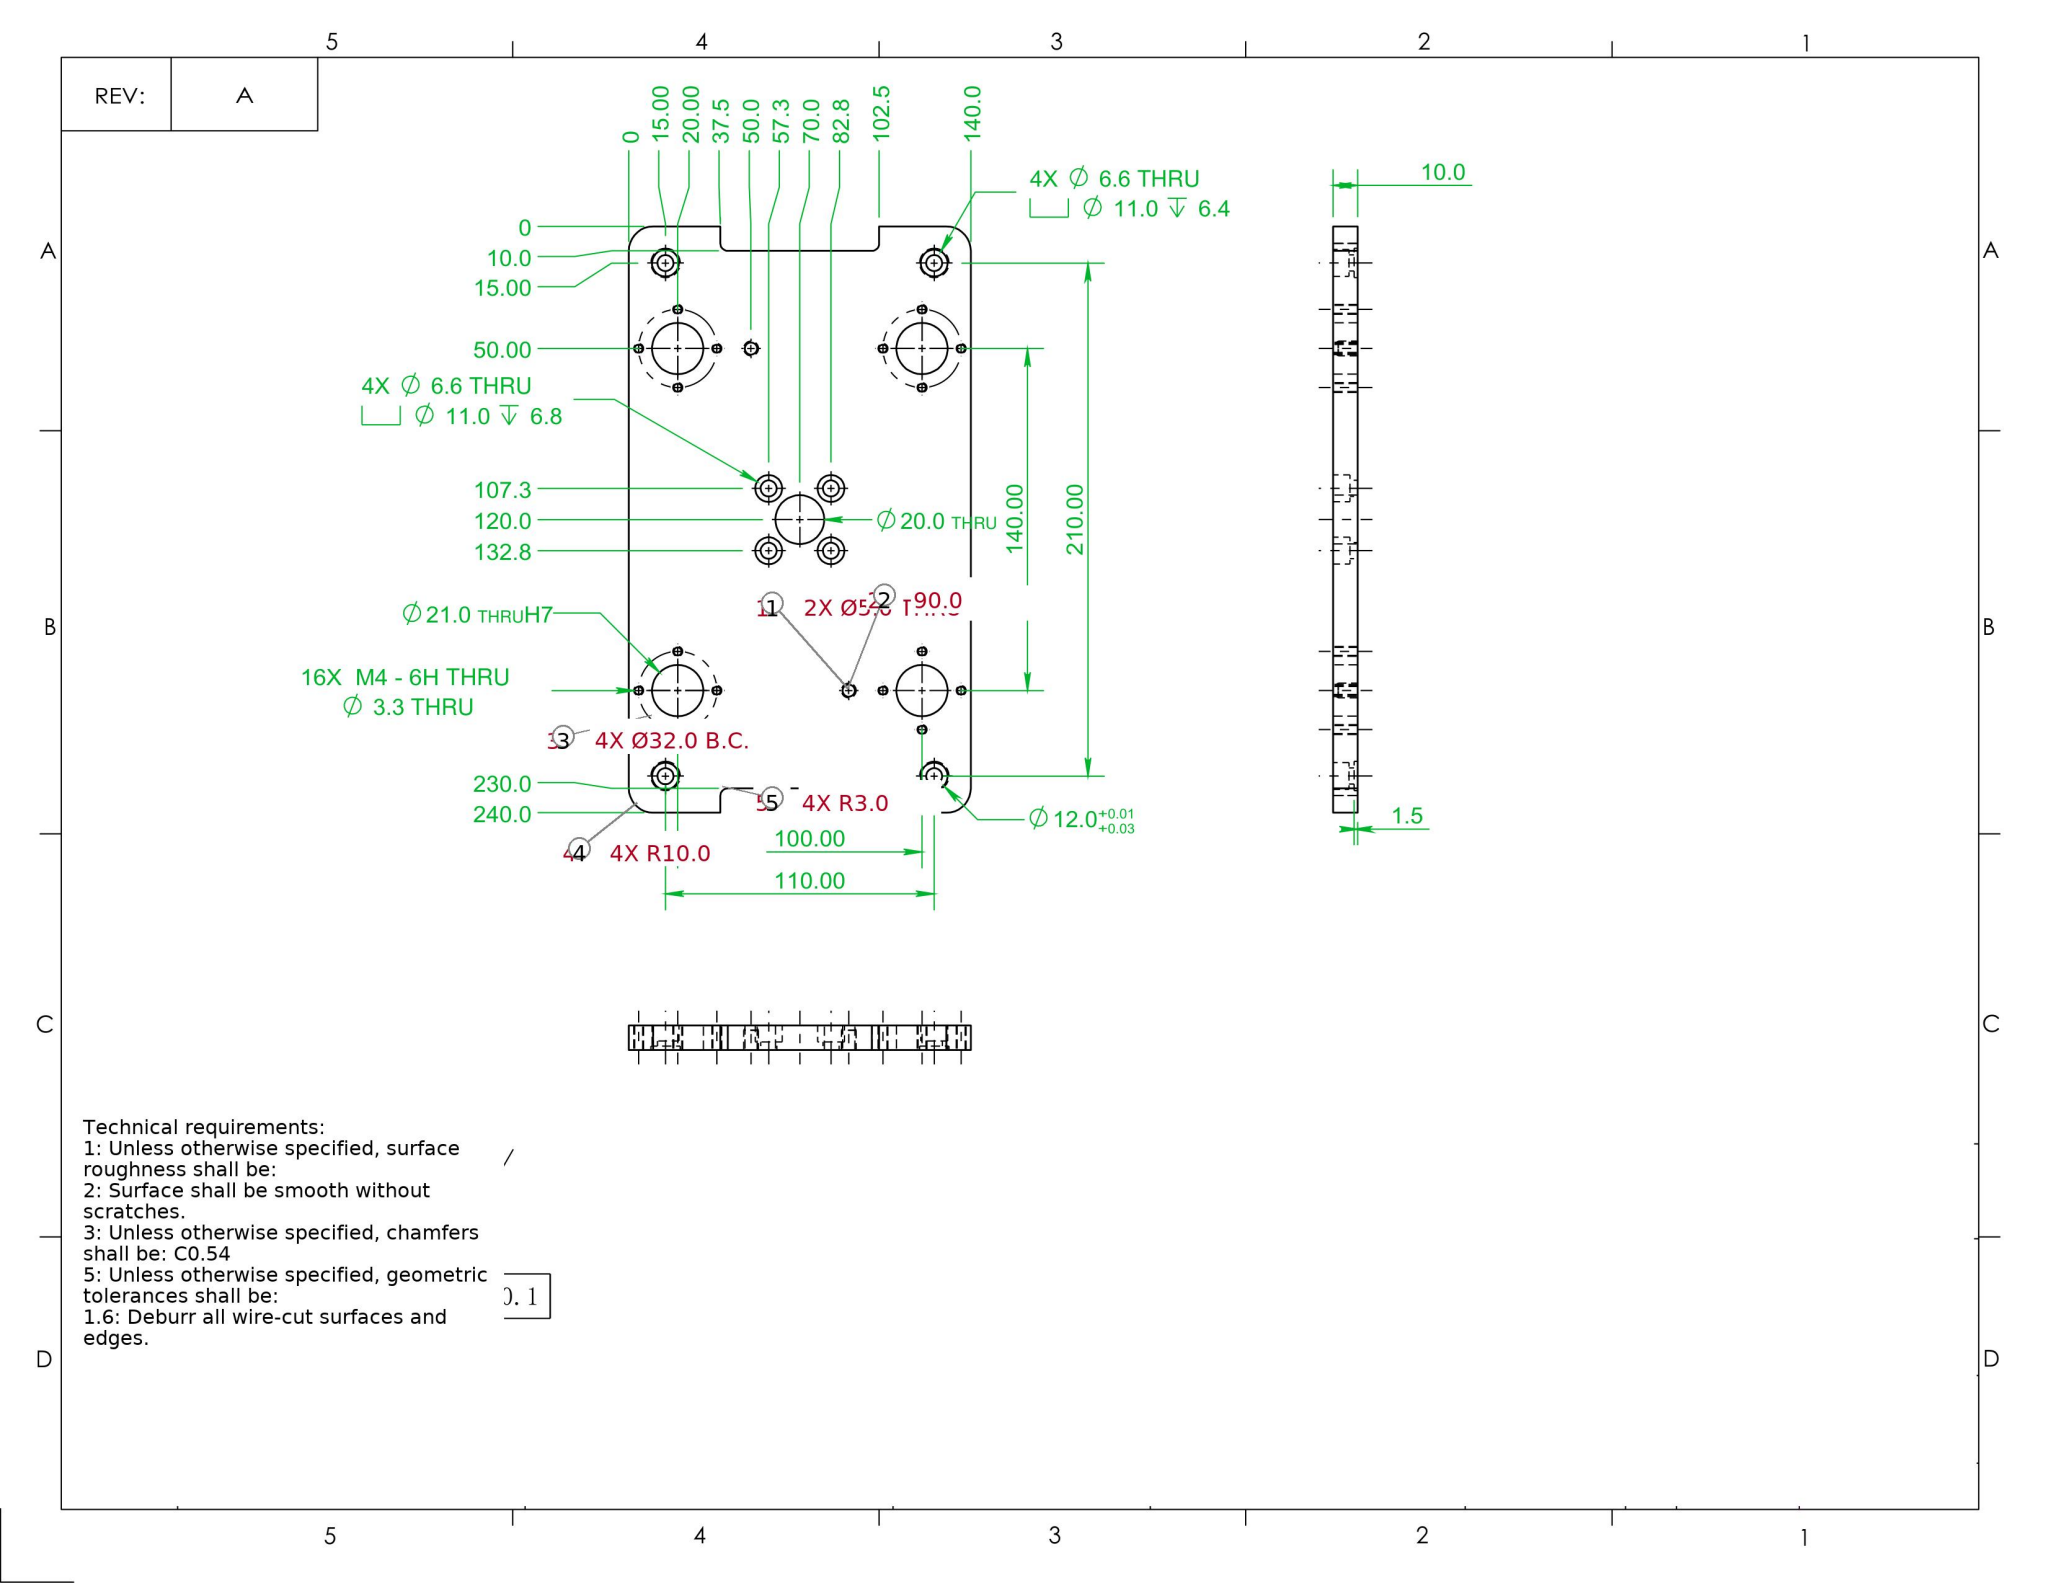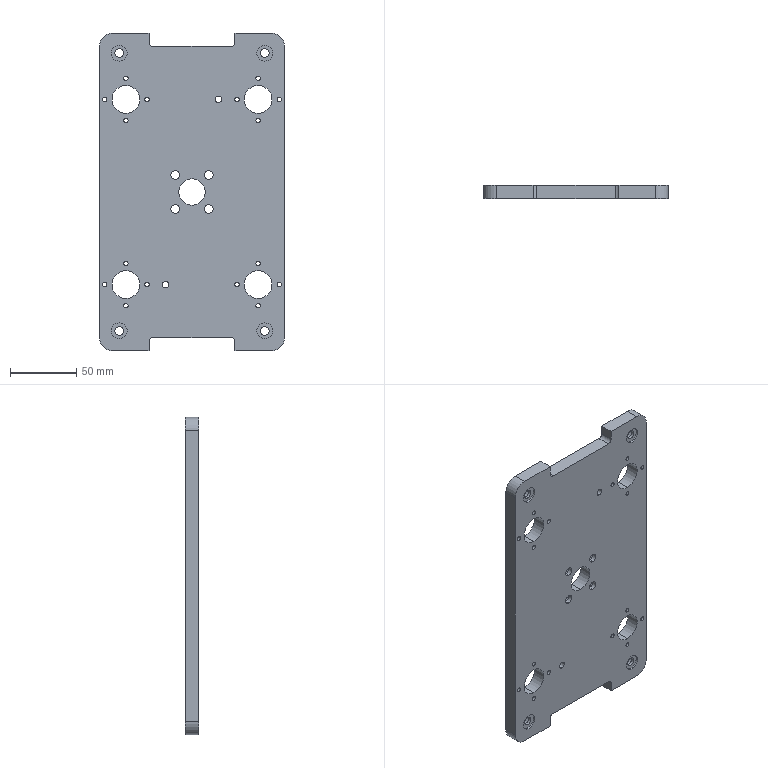Part | SolidWorks | mm | 1 solid | 120 faces | box 140 x 10 x 240 mm | volume 297040 mm3 | cylinder 94 | plane 26 | commonest cylinder face diameters 3.3 x32 11 x16 6.6 x16 12 x8 21 x8 20 x6 5 x4 6 x4
build123d program:
from build123d import *

# Parameters (mm, degrees)
SKETCH1_W                                         = 140
SKETCH1_H                                         = 240
BOSS_EXTRUDE1_DEPTH                               = 10
FILLET1_R                                         = 10
SKETCH2_R                                         = 10.5
CUT_EXTRUDE1_DEPTH                                = 279.029
M4_TAPPED_HOLE1_D                                 = 3.3
M6_HEX_SOCKET_HEAD_CAP_SCREW_CBORE1_D             = 6.6
M6_HEX_SOCKET_HEAD_CAP_SCREW_CBORE1_CBORE_D       = 11
M6_HEX_SOCKET_HEAD_CAP_SCREW_CBORE1_CBORE_DEPTH   = 6.4
SKETCH21_R                                        = 6
CUT_EXTRUDE6_DEPTH                                = 1.5
SKETCH22_R                                        = 10
CUT_EXTRUDE7_DEPTH                                = 279.029
M6_TAPPED_HOLE1_D                                 = 5
M6_TAPPED_HOLE1_DEPTH                             = 13
M6_TAPPED_HOLE1_TIP                               = 1.502
HOLE_SIZE_ACCORDING_TO_HEXAGON_SOCKET_D           = 6.6
HOLE_SIZE_ACCORDING_TO_HEXAGON_SOCKET_CBORE_D     = 11
HOLE_SIZE_ACCORDING_TO_HEXAGON_SOCKET_CBORE_DEPTH = 6.8
SKETCH36_W                                        = 65
SKETCH36_H                                        = 10
CUT_EXTRUDE8_DEPTH                                = 279.029
FILLET2_R                                         = 3


with BuildPart() as part:
    # Sketch1 → Boss-Extrude1 (new body)
    with BuildSketch(Plane(origin=(0, 0, 0), x_dir=(1, 0, 0), z_dir=(0, 1, 0))):
        with Locations((70, 120)):
            Rectangle(SKETCH1_W, SKETCH1_H)
    extrude(amount=BOSS_EXTRUDE1_DEPTH)

    # Fillet1
    fillet1_edges = [part.edges().sort_by_distance(p)[0] for p in [
        (0, 5, -240),
        (140, 5, -240),
        (140, 5, 0),
        (0, 5, 0),
    ]]
    fillet(fillet1_edges, radius=FILLET1_R)

    # Sketch2 → Cut-Extrude1 (cut, through all)
    with BuildSketch(Plane.XZ):
        with Locations(Location((20, -50, 0), (0, 0, 270))):
            Circle(SKETCH2_R)
        with Locations(Location((20, -190, 0), (0, 0, 270))):
            Circle(SKETCH2_R)
        with Locations(Location((120, -190, 0), (0, 0, 270))):
            Circle(SKETCH2_R)
        with Locations(Location((120, -50, 0), (0, 0, 270))):
            Circle(SKETCH2_R)
    extrude(amount=-CUT_EXTRUDE1_DEPTH, mode=Mode.SUBTRACT)

    # M4 Tapped Hole1 (through all)
    with Locations(Plane(origin=(0, 10, 0), x_dir=(1, 0, 0), z_dir=(0, 1, 0))):
        with Locations((36, 190), (4, 190), (104, 190), (136, 190), (136, 50), (104, 50), (36, 50), (4, 50), (20, 206), (20, 174), (20, 66), (20, 34), (120, 66), (120, 34), (120, 206), (120, 174)):
            Hole(M4_TAPPED_HOLE1_D / 2)

    # M6 Hex Socket Head Cap Screw CBORE1 (through all)
    with Locations(Plane(origin=(0, 10, 0), x_dir=(1, 0, 0), z_dir=(0, 1, 0))):
        with Locations((15, 225), (125, 225), (15, 15), (125, 15)):
            CounterBoreHole(M6_HEX_SOCKET_HEAD_CAP_SCREW_CBORE1_D / 2, M6_HEX_SOCKET_HEAD_CAP_SCREW_CBORE1_CBORE_D / 2, M6_HEX_SOCKET_HEAD_CAP_SCREW_CBORE1_CBORE_DEPTH)

    # Sketch21 → Cut-Extrude6 (cut)
    with BuildSketch(Plane.XZ):
        with Locations(Location((15, -15, 0), (0, 0, 270))):
            Circle(SKETCH21_R)
        with Locations(Location((125, -15, 0), (0, 0, 270))):
            Circle(SKETCH21_R)
        with Locations(Location((15, -225, 0), (0, 0, 270))):
            Circle(SKETCH21_R)
        with Locations(Location((125, -225, 0), (0, 0, 270))):
            Circle(SKETCH21_R)
    extrude(amount=-CUT_EXTRUDE6_DEPTH, mode=Mode.SUBTRACT)

    # Sketch22 → Cut-Extrude7 (cut, through all)
    with BuildSketch(Plane.XZ):
        with Locations(Location((70, -120, 0), (0, 0, 270))):
            Circle(SKETCH22_R)
    extrude(amount=-CUT_EXTRUDE7_DEPTH, mode=Mode.SUBTRACT)

    # M6 Tapped Hole1
    with Locations(Plane(origin=(0, 0, 0), x_dir=(-1, 0, 0), z_dir=(0, -1, 0))):
        with Locations((-50, 190), (-90, 50)):
            Hole(M6_TAPPED_HOLE1_D / 2, depth=M6_TAPPED_HOLE1_DEPTH)
            with Locations((0, 0, -(M6_TAPPED_HOLE1_DEPTH + M6_TAPPED_HOLE1_TIP / 2))):  # 118° drill point
                Cone(0, M6_TAPPED_HOLE1_D / 2, M6_TAPPED_HOLE1_TIP, mode=Mode.SUBTRACT)

    # Hole Size _ according to_ Hexagon Socket (through all)
    with Locations(Plane(origin=(0, 10, 0), x_dir=(1, 0, 0), z_dir=(0, 1, 0))):
        with Locations((82.75, 107.25), (57.25, 132.75), (57.25, 107.25), (82.75, 132.75)):
            CounterBoreHole(HOLE_SIZE_ACCORDING_TO_HEXAGON_SOCKET_D / 2, HOLE_SIZE_ACCORDING_TO_HEXAGON_SOCKET_CBORE_D / 2, HOLE_SIZE_ACCORDING_TO_HEXAGON_SOCKET_CBORE_DEPTH)

    # Sketch36 → Cut-Extrude8 (cut, through all)
    with BuildSketch(Plane(origin=(0, 10, 0), x_dir=(1, 0, 0), z_dir=(0, 1, 0))):
        with Locations((70, 235)):
            Rectangle(SKETCH36_W, SKETCH36_H)
        with Locations((70, 5)):
            Rectangle(SKETCH36_W, SKETCH36_H)
    extrude(amount=-CUT_EXTRUDE8_DEPTH, mode=Mode.SUBTRACT)

    # Fillet2
    fillet2_edges = [part.edges().sort_by_distance(p)[0] for p in [
        (37.5, 5, -230),
        (102.5, 5, -230),
        (37.5, 5, -10),
        (102.5, 5, -10),
    ]]
    fillet(fillet2_edges, radius=FILLET2_R)


solid = part.part